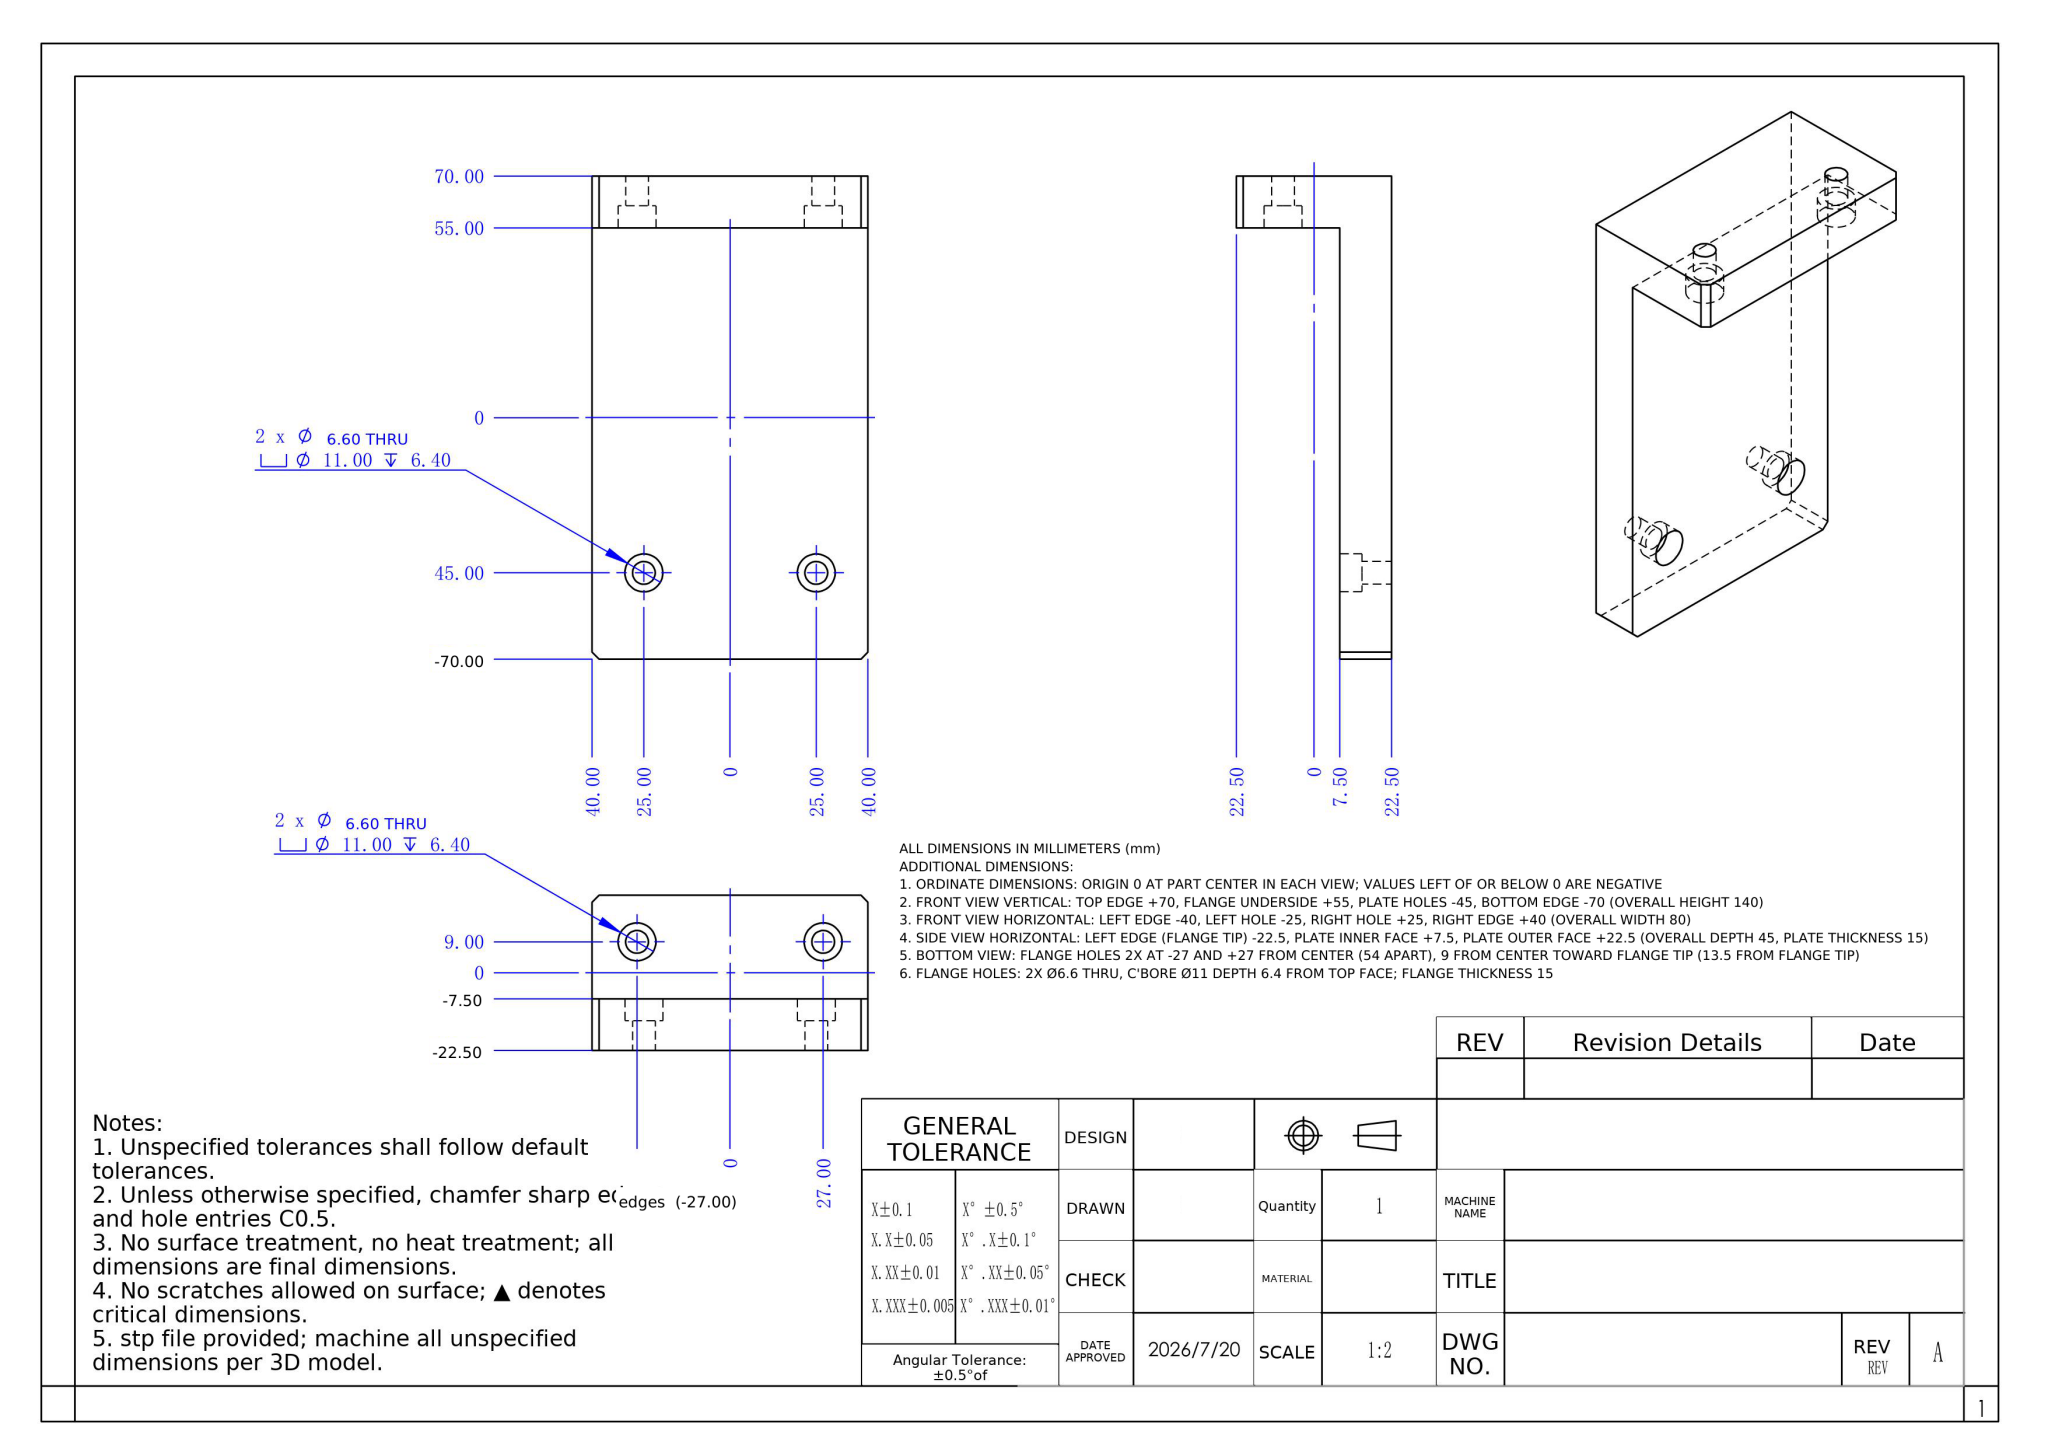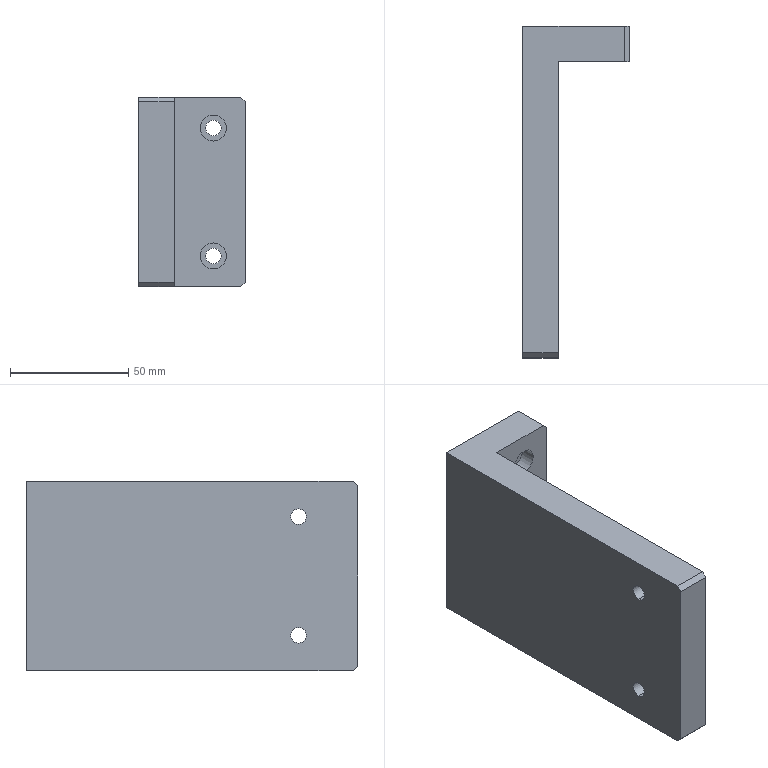Part | NX | mm | 1 solid | 32 faces | box 45 x 140 x 80 mm | volume 200270 mm3 | cylinder 16 | plane 16 | commonest cylinder face diameters 11 x8 6.6 x8
STEP:
#1=CARTESIAN_POINT('',(8.6,25.,20.5));
#2=VERTEX_POINT('',#1);
#3=CARTESIAN_POINT('',(8.6,25.,9.5));
#4=VERTEX_POINT('',#3);
#5=CARTESIAN_POINT('',(8.6,25.,15.));
#6=DIRECTION('',(1.,0.,0.));
#7=DIRECTION('',(0.,0.,-1.));
#8=AXIS2_PLACEMENT_3D('',#5,#6,#7);
#9=CIRCLE('',#8,5.5);
#10=EDGE_CURVE('',#2,#4,#9,.T.);
#11=ORIENTED_EDGE('',*,*,#10,.F.);
#12=CARTESIAN_POINT('',(15.,25.,20.5));
#13=VERTEX_POINT('',#12);
#14=CARTESIAN_POINT('',(15.,25.,20.5));
#15=DIRECTION('',(1.,0.,0.));
#16=VECTOR('',#15,1000.);
#17=LINE('',#14,#16);
#18=EDGE_CURVE('',#2,#13,#17,.T.);
#19=ORIENTED_EDGE('',*,*,#18,.T.);
#20=CARTESIAN_POINT('',(15.,25.,9.5));
#21=VERTEX_POINT('',#20);
#22=CARTESIAN_POINT('',(15.,25.,15.));
#23=DIRECTION('',(1.,0.,0.));
#24=DIRECTION('',(0.,0.,-1.));
#25=AXIS2_PLACEMENT_3D('',#22,#23,#24);
#26=CIRCLE('',#25,5.5);
#27=EDGE_CURVE('',#13,#21,#26,.T.);
#28=ORIENTED_EDGE('',*,*,#27,.T.);
#29=CARTESIAN_POINT('',(15.,25.,9.5));
#30=DIRECTION('',(1.,0.,0.));
#31=VECTOR('',#30,1000.);
#32=LINE('',#29,#31);
#33=EDGE_CURVE('',#4,#21,#32,.T.);
#34=ORIENTED_EDGE('',*,*,#33,.F.);
#35=EDGE_LOOP('',(#11,#19,#28,#34));
#36=FACE_OUTER_BOUND('',#35,.T.);
#37=CARTESIAN_POINT('',(15.,25.,15.));
#38=DIRECTION('',(1.,0.,0.));
#39=DIRECTION('',(0.,0.,-1.));
#40=AXIS2_PLACEMENT_3D('',#37,#38,#39);
#41=CYLINDRICAL_SURFACE('',#40,5.5);
#42=ADVANCED_FACE('',(#36),#41,.F.);
#43=CARTESIAN_POINT('',(0.,25.,18.3));
#44=VERTEX_POINT('',#43);
#45=CARTESIAN_POINT('',(0.,25.,11.7));
#46=VERTEX_POINT('',#45);
#47=CARTESIAN_POINT('',(0.,25.,15.));
#48=DIRECTION('',(1.,0.,0.));
#49=DIRECTION('',(0.,0.,-1.));
#50=AXIS2_PLACEMENT_3D('',#47,#48,#49);
#51=CIRCLE('',#50,3.3);
#52=EDGE_CURVE('',#44,#46,#51,.T.);
#53=ORIENTED_EDGE('',*,*,#52,.F.);
#54=CARTESIAN_POINT('',(8.6,25.,18.3));
#55=VERTEX_POINT('',#54);
#56=CARTESIAN_POINT('',(15.,25.,18.3));
#57=DIRECTION('',(1.,0.,0.));
#58=VECTOR('',#57,1000.);
#59=LINE('',#56,#58);
#60=EDGE_CURVE('',#44,#55,#59,.T.);
#61=ORIENTED_EDGE('',*,*,#60,.T.);
#62=CARTESIAN_POINT('',(8.6,25.,11.7));
#63=VERTEX_POINT('',#62);
#64=CARTESIAN_POINT('',(8.6,25.,15.));
#65=DIRECTION('',(1.,0.,0.));
#66=DIRECTION('',(0.,0.,-1.));
#67=AXIS2_PLACEMENT_3D('',#64,#65,#66);
#68=CIRCLE('',#67,3.3);
#69=EDGE_CURVE('',#55,#63,#68,.T.);
#70=ORIENTED_EDGE('',*,*,#69,.T.);
#71=CARTESIAN_POINT('',(15.,25.,11.7));
#72=DIRECTION('',(1.,0.,0.));
#73=VECTOR('',#72,1000.);
#74=LINE('',#71,#73);
#75=EDGE_CURVE('',#46,#63,#74,.T.);
#76=ORIENTED_EDGE('',*,*,#75,.F.);
#77=EDGE_LOOP('',(#53,#61,#70,#76));
#78=FACE_OUTER_BOUND('',#77,.T.);
#79=CARTESIAN_POINT('',(15.,25.,15.));
#80=DIRECTION('',(1.,0.,0.));
#81=DIRECTION('',(0.,0.,-1.));
#82=AXIS2_PLACEMENT_3D('',#79,#80,#81);
#83=CYLINDRICAL_SURFACE('',#82,3.3);
#84=ADVANCED_FACE('',(#78),#83,.F.);
#85=CARTESIAN_POINT('',(8.6,25.,70.5));
#86=VERTEX_POINT('',#85);
#87=CARTESIAN_POINT('',(8.6,25.,59.5));
#88=VERTEX_POINT('',#87);
#89=CARTESIAN_POINT('',(8.6,25.,65.));
#90=DIRECTION('',(1.,0.,0.));
#91=DIRECTION('',(0.,0.,-1.));
#92=AXIS2_PLACEMENT_3D('',#89,#90,#91);
#93=CIRCLE('',#92,5.5);
#94=EDGE_CURVE('',#86,#88,#93,.T.);
#95=ORIENTED_EDGE('',*,*,#94,.F.);
#96=CARTESIAN_POINT('',(15.,25.,70.5));
#97=VERTEX_POINT('',#96);
#98=CARTESIAN_POINT('',(15.,25.,70.5));
#99=DIRECTION('',(1.,0.,0.));
#100=VECTOR('',#99,1000.);
#101=LINE('',#98,#100);
#102=EDGE_CURVE('',#86,#97,#101,.T.);
#103=ORIENTED_EDGE('',*,*,#102,.T.);
#104=CARTESIAN_POINT('',(15.,25.,59.5));
#105=VERTEX_POINT('',#104);
#106=CARTESIAN_POINT('',(15.,25.,65.));
#107=DIRECTION('',(1.,0.,0.));
#108=DIRECTION('',(0.,0.,-1.));
#109=AXIS2_PLACEMENT_3D('',#106,#107,#108);
#110=CIRCLE('',#109,5.5);
#111=EDGE_CURVE('',#97,#105,#110,.T.);
#112=ORIENTED_EDGE('',*,*,#111,.T.);
#113=CARTESIAN_POINT('',(15.,25.,59.5));
#114=DIRECTION('',(1.,0.,0.));
#115=VECTOR('',#114,1000.);
#116=LINE('',#113,#115);
#117=EDGE_CURVE('',#88,#105,#116,.T.);
#118=ORIENTED_EDGE('',*,*,#117,.F.);
#119=EDGE_LOOP('',(#95,#103,#112,#118));
#120=FACE_OUTER_BOUND('',#119,.T.);
#121=CARTESIAN_POINT('',(15.,25.,65.));
#122=DIRECTION('',(1.,0.,0.));
#123=DIRECTION('',(0.,0.,-1.));
#124=AXIS2_PLACEMENT_3D('',#121,#122,#123);
#125=CYLINDRICAL_SURFACE('',#124,5.5);
#126=ADVANCED_FACE('',(#120),#125,.F.);
#127=CARTESIAN_POINT('',(0.,25.,68.3));
#128=VERTEX_POINT('',#127);
#129=CARTESIAN_POINT('',(0.,25.,61.7));
#130=VERTEX_POINT('',#129);
#131=CARTESIAN_POINT('',(0.,25.,65.));
#132=DIRECTION('',(1.,0.,0.));
#133=DIRECTION('',(0.,0.,-1.));
#134=AXIS2_PLACEMENT_3D('',#131,#132,#133);
#135=CIRCLE('',#134,3.3);
#136=EDGE_CURVE('',#128,#130,#135,.T.);
#137=ORIENTED_EDGE('',*,*,#136,.F.);
#138=CARTESIAN_POINT('',(8.6,25.,68.3));
#139=VERTEX_POINT('',#138);
#140=CARTESIAN_POINT('',(15.,25.,68.3));
#141=DIRECTION('',(1.,0.,0.));
#142=VECTOR('',#141,1000.);
#143=LINE('',#140,#142);
#144=EDGE_CURVE('',#128,#139,#143,.T.);
#145=ORIENTED_EDGE('',*,*,#144,.T.);
#146=CARTESIAN_POINT('',(8.6,25.,61.7));
#147=VERTEX_POINT('',#146);
#148=CARTESIAN_POINT('',(8.6,25.,65.));
#149=DIRECTION('',(1.,0.,0.));
#150=DIRECTION('',(0.,0.,-1.));
#151=AXIS2_PLACEMENT_3D('',#148,#149,#150);
#152=CIRCLE('',#151,3.3);
#153=EDGE_CURVE('',#139,#147,#152,.T.);
#154=ORIENTED_EDGE('',*,*,#153,.T.);
#155=CARTESIAN_POINT('',(15.,25.,61.7));
#156=DIRECTION('',(1.,0.,0.));
#157=VECTOR('',#156,1000.);
#158=LINE('',#155,#157);
#159=EDGE_CURVE('',#130,#147,#158,.T.);
#160=ORIENTED_EDGE('',*,*,#159,.F.);
#161=EDGE_LOOP('',(#137,#145,#154,#160));
#162=FACE_OUTER_BOUND('',#161,.T.);
#163=CARTESIAN_POINT('',(15.,25.,65.));
#164=DIRECTION('',(1.,0.,0.));
#165=DIRECTION('',(0.,0.,-1.));
#166=AXIS2_PLACEMENT_3D('',#163,#164,#165);
#167=CYLINDRICAL_SURFACE('',#166,3.3);
#168=ADVANCED_FACE('',(#162),#167,.F.);
#169=CARTESIAN_POINT('',(31.5,131.4,18.5));
#170=VERTEX_POINT('',#169);
#171=CARTESIAN_POINT('',(31.5,131.4,7.5));
#172=VERTEX_POINT('',#171);
#173=CARTESIAN_POINT('',(31.5,131.4,13.));
#174=DIRECTION('',(0.,-1.,0.));
#175=DIRECTION('',(0.,0.,-1.));
#176=AXIS2_PLACEMENT_3D('',#173,#174,#175);
#177=CIRCLE('',#176,5.5);
#178=EDGE_CURVE('',#170,#172,#177,.T.);
#179=ORIENTED_EDGE('',*,*,#178,.F.);
#180=CARTESIAN_POINT('',(31.5,125.,18.5));
#181=VERTEX_POINT('',#180);
#182=CARTESIAN_POINT('',(31.5,125.,18.5));
#183=DIRECTION('',(0.,-1.,0.));
#184=VECTOR('',#183,1000.);
#185=LINE('',#182,#184);
#186=EDGE_CURVE('',#170,#181,#185,.T.);
#187=ORIENTED_EDGE('',*,*,#186,.T.);
#188=CARTESIAN_POINT('',(31.5,125.,7.5));
#189=VERTEX_POINT('',#188);
#190=CARTESIAN_POINT('',(31.5,125.,13.));
#191=DIRECTION('',(0.,-1.,0.));
#192=DIRECTION('',(0.,0.,-1.));
#193=AXIS2_PLACEMENT_3D('',#190,#191,#192);
#194=CIRCLE('',#193,5.5);
#195=EDGE_CURVE('',#181,#189,#194,.T.);
#196=ORIENTED_EDGE('',*,*,#195,.T.);
#197=CARTESIAN_POINT('',(31.5,125.,7.5));
#198=DIRECTION('',(0.,-1.,0.));
#199=VECTOR('',#198,1000.);
#200=LINE('',#197,#199);
#201=EDGE_CURVE('',#172,#189,#200,.T.);
#202=ORIENTED_EDGE('',*,*,#201,.F.);
#203=EDGE_LOOP('',(#179,#187,#196,#202));
#204=FACE_OUTER_BOUND('',#203,.T.);
#205=CARTESIAN_POINT('',(31.5,125.,13.));
#206=DIRECTION('',(0.,-1.,0.));
#207=DIRECTION('',(0.,0.,-1.));
#208=AXIS2_PLACEMENT_3D('',#205,#206,#207);
#209=CYLINDRICAL_SURFACE('',#208,5.5);
#210=ADVANCED_FACE('',(#204),#209,.F.);
#211=CARTESIAN_POINT('',(31.5,140.,16.3));
#212=VERTEX_POINT('',#211);
#213=CARTESIAN_POINT('',(31.5,140.,9.7));
#214=VERTEX_POINT('',#213);
#215=CARTESIAN_POINT('',(31.5,140.,13.));
#216=DIRECTION('',(0.,-1.,0.));
#217=DIRECTION('',(0.,0.,-1.));
#218=AXIS2_PLACEMENT_3D('',#215,#216,#217);
#219=CIRCLE('',#218,3.3);
#220=EDGE_CURVE('',#212,#214,#219,.T.);
#221=ORIENTED_EDGE('',*,*,#220,.F.);
#222=CARTESIAN_POINT('',(31.5,131.4,16.3));
#223=VERTEX_POINT('',#222);
#224=CARTESIAN_POINT('',(31.5,125.,16.3));
#225=DIRECTION('',(0.,-1.,0.));
#226=VECTOR('',#225,1000.);
#227=LINE('',#224,#226);
#228=EDGE_CURVE('',#212,#223,#227,.T.);
#229=ORIENTED_EDGE('',*,*,#228,.T.);
#230=CARTESIAN_POINT('',(31.5,131.4,9.7));
#231=VERTEX_POINT('',#230);
#232=CARTESIAN_POINT('',(31.5,131.4,13.));
#233=DIRECTION('',(0.,-1.,0.));
#234=DIRECTION('',(0.,0.,-1.));
#235=AXIS2_PLACEMENT_3D('',#232,#233,#234);
#236=CIRCLE('',#235,3.3);
#237=EDGE_CURVE('',#223,#231,#236,.T.);
#238=ORIENTED_EDGE('',*,*,#237,.T.);
#239=CARTESIAN_POINT('',(31.5,125.,9.7));
#240=DIRECTION('',(0.,-1.,0.));
#241=VECTOR('',#240,1000.);
#242=LINE('',#239,#241);
#243=EDGE_CURVE('',#214,#231,#242,.T.);
#244=ORIENTED_EDGE('',*,*,#243,.F.);
#245=EDGE_LOOP('',(#221,#229,#238,#244));
#246=FACE_OUTER_BOUND('',#245,.T.);
#247=CARTESIAN_POINT('',(31.5,125.,13.));
#248=DIRECTION('',(0.,-1.,0.));
#249=DIRECTION('',(0.,0.,-1.));
#250=AXIS2_PLACEMENT_3D('',#247,#248,#249);
#251=CYLINDRICAL_SURFACE('',#250,3.3);
#252=ADVANCED_FACE('',(#246),#251,.F.);
#253=CARTESIAN_POINT('',(31.5,131.4,72.5));
#254=VERTEX_POINT('',#253);
#255=CARTESIAN_POINT('',(31.5,131.4,61.5));
#256=VERTEX_POINT('',#255);
#257=CARTESIAN_POINT('',(31.5,131.4,67.));
#258=DIRECTION('',(0.,-1.,0.));
#259=DIRECTION('',(0.,0.,-1.));
#260=AXIS2_PLACEMENT_3D('',#257,#258,#259);
#261=CIRCLE('',#260,5.5);
#262=EDGE_CURVE('',#254,#256,#261,.T.);
#263=ORIENTED_EDGE('',*,*,#262,.F.);
#264=CARTESIAN_POINT('',(31.5,125.,72.5));
#265=VERTEX_POINT('',#264);
#266=CARTESIAN_POINT('',(31.5,125.,72.5));
#267=DIRECTION('',(0.,-1.,0.));
#268=VECTOR('',#267,1000.);
#269=LINE('',#266,#268);
#270=EDGE_CURVE('',#254,#265,#269,.T.);
#271=ORIENTED_EDGE('',*,*,#270,.T.);
#272=CARTESIAN_POINT('',(31.5,125.,61.5));
#273=VERTEX_POINT('',#272);
#274=CARTESIAN_POINT('',(31.5,125.,67.));
#275=DIRECTION('',(0.,-1.,0.));
#276=DIRECTION('',(0.,0.,-1.));
#277=AXIS2_PLACEMENT_3D('',#274,#275,#276);
#278=CIRCLE('',#277,5.5);
#279=EDGE_CURVE('',#265,#273,#278,.T.);
#280=ORIENTED_EDGE('',*,*,#279,.T.);
#281=CARTESIAN_POINT('',(31.5,125.,61.5));
#282=DIRECTION('',(0.,-1.,0.));
#283=VECTOR('',#282,1000.);
#284=LINE('',#281,#283);
#285=EDGE_CURVE('',#256,#273,#284,.T.);
#286=ORIENTED_EDGE('',*,*,#285,.F.);
#287=EDGE_LOOP('',(#263,#271,#280,#286));
#288=FACE_OUTER_BOUND('',#287,.T.);
#289=CARTESIAN_POINT('',(31.5,125.,67.));
#290=DIRECTION('',(0.,-1.,0.));
#291=DIRECTION('',(0.,0.,-1.));
#292=AXIS2_PLACEMENT_3D('',#289,#290,#291);
#293=CYLINDRICAL_SURFACE('',#292,5.5);
#294=ADVANCED_FACE('',(#288),#293,.F.);
#295=CARTESIAN_POINT('',(31.5,140.,70.3));
#296=VERTEX_POINT('',#295);
#297=CARTESIAN_POINT('',(31.5,140.,63.7));
#298=VERTEX_POINT('',#297);
#299=CARTESIAN_POINT('',(31.5,140.,67.));
#300=DIRECTION('',(0.,-1.,0.));
#301=DIRECTION('',(0.,0.,-1.));
#302=AXIS2_PLACEMENT_3D('',#299,#300,#301);
#303=CIRCLE('',#302,3.3);
#304=EDGE_CURVE('',#296,#298,#303,.T.);
#305=ORIENTED_EDGE('',*,*,#304,.F.);
#306=CARTESIAN_POINT('',(31.5,131.4,70.3));
#307=VERTEX_POINT('',#306);
#308=CARTESIAN_POINT('',(31.5,125.,70.3));
#309=DIRECTION('',(0.,-1.,0.));
#310=VECTOR('',#309,1000.);
#311=LINE('',#308,#310);
#312=EDGE_CURVE('',#296,#307,#311,.T.);
#313=ORIENTED_EDGE('',*,*,#312,.T.);
#314=CARTESIAN_POINT('',(31.5,131.4,63.7));
#315=VERTEX_POINT('',#314);
#316=CARTESIAN_POINT('',(31.5,131.4,67.));
#317=DIRECTION('',(0.,-1.,0.));
#318=DIRECTION('',(0.,0.,-1.));
#319=AXIS2_PLACEMENT_3D('',#316,#317,#318);
#320=CIRCLE('',#319,3.3);
#321=EDGE_CURVE('',#307,#315,#320,.T.);
#322=ORIENTED_EDGE('',*,*,#321,.T.);
#323=CARTESIAN_POINT('',(31.5,125.,63.7));
#324=DIRECTION('',(0.,-1.,0.));
#325=VECTOR('',#324,1000.);
#326=LINE('',#323,#325);
#327=EDGE_CURVE('',#298,#315,#326,.T.);
#328=ORIENTED_EDGE('',*,*,#327,.F.);
#329=EDGE_LOOP('',(#305,#313,#322,#328));
#330=FACE_OUTER_BOUND('',#329,.T.);
#331=CARTESIAN_POINT('',(31.5,125.,67.));
#332=DIRECTION('',(0.,-1.,0.));
#333=DIRECTION('',(0.,0.,-1.));
#334=AXIS2_PLACEMENT_3D('',#331,#332,#333);
#335=CYLINDRICAL_SURFACE('',#334,3.3);
#336=ADVANCED_FACE('',(#330),#335,.F.);
#337=CARTESIAN_POINT('',(0.,2.,80.));
#338=VERTEX_POINT('',#337);
#339=CARTESIAN_POINT('',(0.,140.,80.));
#340=VERTEX_POINT('',#339);
#341=CARTESIAN_POINT('',(0.,0.,80.));
#342=DIRECTION('',(0.,1.,0.));
#343=VECTOR('',#342,1000.);
#344=LINE('',#341,#343);
#345=EDGE_CURVE('',#338,#340,#344,.T.);
#346=ORIENTED_EDGE('',*,*,#345,.F.);
#347=CARTESIAN_POINT('',(15.,2.,80.));
#348=VERTEX_POINT('',#347);
#349=CARTESIAN_POINT('',(0.,2.,80.));
#350=DIRECTION('',(1.,0.,0.));
#351=VECTOR('',#350,1000.);
#352=LINE('',#349,#351);
#353=EDGE_CURVE('',#338,#348,#352,.T.);
#354=ORIENTED_EDGE('',*,*,#353,.T.);
#355=CARTESIAN_POINT('',(15.,125.,80.));
#356=VERTEX_POINT('',#355);
#357=CARTESIAN_POINT('',(15.,0.,80.));
#358=DIRECTION('',(0.,1.,0.));
#359=VECTOR('',#358,1000.);
#360=LINE('',#357,#359);
#361=EDGE_CURVE('',#348,#356,#360,.T.);
#362=ORIENTED_EDGE('',*,*,#361,.T.);
#363=CARTESIAN_POINT('',(43.,125.,80.));
#364=VERTEX_POINT('',#363);
#365=CARTESIAN_POINT('',(15.,125.,80.));
#366=DIRECTION('',(1.,0.,0.));
#367=VECTOR('',#366,1000.);
#368=LINE('',#365,#367);
#369=EDGE_CURVE('',#356,#364,#368,.T.);
#370=ORIENTED_EDGE('',*,*,#369,.T.);
#371=CARTESIAN_POINT('',(43.,140.,80.));
#372=VERTEX_POINT('',#371);
#373=CARTESIAN_POINT('',(43.,140.,80.));
#374=DIRECTION('',(0.,1.,0.));
#375=VECTOR('',#374,1000.);
#376=LINE('',#373,#375);
#377=EDGE_CURVE('',#364,#372,#376,.T.);
#378=ORIENTED_EDGE('',*,*,#377,.T.);
#379=CARTESIAN_POINT('',(15.,140.,80.));
#380=DIRECTION('',(1.,0.,0.));
#381=VECTOR('',#380,1000.);
#382=LINE('',#379,#381);
#383=EDGE_CURVE('',#340,#372,#382,.T.);
#384=ORIENTED_EDGE('',*,*,#383,.F.);
#385=EDGE_LOOP('',(#346,#354,#362,#370,#378,#384));
#386=FACE_OUTER_BOUND('',#385,.T.);
#387=CARTESIAN_POINT('',(0.,0.,80.));
#388=DIRECTION('',(0.,0.,-1.));
#389=DIRECTION('',(-1.,0.,0.));
#390=AXIS2_PLACEMENT_3D('',#387,#388,#389);
#391=PLANE('',#390);
#392=ADVANCED_FACE('',(#386),#391,.F.);
#393=CARTESIAN_POINT('',(45.,140.,78.));
#394=VERTEX_POINT('',#393);
#395=CARTESIAN_POINT('',(45.,140.,2.));
#396=VERTEX_POINT('',#395);
#397=CARTESIAN_POINT('',(45.,140.,80.));
#398=DIRECTION('',(0.,0.,-1.));
#399=VECTOR('',#398,1000.);
#400=LINE('',#397,#399);
#401=EDGE_CURVE('',#394,#396,#400,.T.);
#402=ORIENTED_EDGE('',*,*,#401,.F.);
#403=CARTESIAN_POINT('',(45.,125.,78.));
#404=VERTEX_POINT('',#403);
#405=CARTESIAN_POINT('',(45.,125.,78.));
#406=DIRECTION('',(0.,-1.,0.));
#407=VECTOR('',#406,1000.);
#408=LINE('',#405,#407);
#409=EDGE_CURVE('',#394,#404,#408,.T.);
#410=ORIENTED_EDGE('',*,*,#409,.T.);
#411=CARTESIAN_POINT('',(45.,125.,2.));
#412=VERTEX_POINT('',#411);
#413=CARTESIAN_POINT('',(45.,125.,80.));
#414=DIRECTION('',(0.,0.,-1.));
#415=VECTOR('',#414,1000.);
#416=LINE('',#413,#415);
#417=EDGE_CURVE('',#404,#412,#416,.T.);
#418=ORIENTED_EDGE('',*,*,#417,.T.);
#419=CARTESIAN_POINT('',(45.,140.,2.));
#420=DIRECTION('',(0.,1.,0.));
#421=VECTOR('',#420,1000.);
#422=LINE('',#419,#421);
#423=EDGE_CURVE('',#412,#396,#422,.T.);
#424=ORIENTED_EDGE('',*,*,#423,.T.);
#425=EDGE_LOOP('',(#402,#410,#418,#424));
#426=FACE_OUTER_BOUND('',#425,.T.);
#427=CARTESIAN_POINT('',(45.,140.,80.));
#428=DIRECTION('',(1.,0.,0.));
#429=DIRECTION('',(0.,0.,-1.));
#430=AXIS2_PLACEMENT_3D('',#427,#428,#429);
#431=PLANE('',#430);
#432=ADVANCED_FACE('',(#426),#431,.T.);
#433=CARTESIAN_POINT('',(15.,2.,0.));
#434=VERTEX_POINT('',#433);
#435=CARTESIAN_POINT('',(15.,125.,0.));
#436=VERTEX_POINT('',#435);
#437=CARTESIAN_POINT('',(15.,0.,0.));
#438=DIRECTION('',(0.,1.,0.));
#439=VECTOR('',#438,1000.);
#440=LINE('',#437,#439);
#441=EDGE_CURVE('',#434,#436,#440,.T.);
#442=ORIENTED_EDGE('',*,*,#441,.F.);
#443=CARTESIAN_POINT('',(0.,2.,0.));
#444=VERTEX_POINT('',#443);
#445=CARTESIAN_POINT('',(0.,2.,0.));
#446=DIRECTION('',(-1.,0.,0.));
#447=VECTOR('',#446,1000.);
#448=LINE('',#445,#447);
#449=EDGE_CURVE('',#434,#444,#448,.T.);
#450=ORIENTED_EDGE('',*,*,#449,.T.);
#451=CARTESIAN_POINT('',(0.,140.,0.));
#452=VERTEX_POINT('',#451);
#453=CARTESIAN_POINT('',(0.,0.,0.));
#454=DIRECTION('',(0.,1.,0.));
#455=VECTOR('',#454,1000.);
#456=LINE('',#453,#455);
#457=EDGE_CURVE('',#444,#452,#456,.T.);
#458=ORIENTED_EDGE('',*,*,#457,.T.);
#459=CARTESIAN_POINT('',(43.,140.,0.));
#460=VERTEX_POINT('',#459);
#461=CARTESIAN_POINT('',(15.,140.,0.));
#462=DIRECTION('',(1.,0.,0.));
#463=VECTOR('',#462,1000.);
#464=LINE('',#461,#463);
#465=EDGE_CURVE('',#452,#460,#464,.T.);
#466=ORIENTED_EDGE('',*,*,#465,.T.);
#467=CARTESIAN_POINT('',(43.,125.,0.));
#468=VERTEX_POINT('',#467);
#469=CARTESIAN_POINT('',(43.,0.,0.));
#470=DIRECTION('',(0.,-1.,0.));
#471=VECTOR('',#470,1000.);
#472=LINE('',#469,#471);
#473=EDGE_CURVE('',#460,#468,#472,.T.);
#474=ORIENTED_EDGE('',*,*,#473,.T.);
#475=CARTESIAN_POINT('',(15.,125.,0.));
#476=DIRECTION('',(1.,0.,0.));
#477=VECTOR('',#476,1000.);
#478=LINE('',#475,#477);
#479=EDGE_CURVE('',#436,#468,#478,.T.);
#480=ORIENTED_EDGE('',*,*,#479,.F.);
#481=EDGE_LOOP('',(#442,#450,#458,#466,#474,#480));
#482=FACE_OUTER_BOUND('',#481,.T.);
#483=CARTESIAN_POINT('',(0.,0.,0.));
#484=DIRECTION('',(0.,0.,-1.));
#485=DIRECTION('',(-1.,0.,0.));
#486=AXIS2_PLACEMENT_3D('',#483,#484,#485);
#487=PLANE('',#486);
#488=ADVANCED_FACE('',(#482),#487,.T.);
#489=CARTESIAN_POINT('',(31.5,125.,13.));
#490=DIRECTION('',(0.,-1.,0.));
#491=DIRECTION('',(0.,0.,-1.));
#492=AXIS2_PLACEMENT_3D('',#489,#490,#491);
#493=CIRCLE('',#492,5.5);
#494=EDGE_CURVE('',#189,#181,#493,.T.);
#495=ORIENTED_EDGE('',*,*,#494,.F.);
#496=ORIENTED_EDGE('',*,*,#195,.F.);
#497=EDGE_LOOP('',(#495,#496));
#498=FACE_BOUND('',#497,.T.);
#499=CARTESIAN_POINT('',(31.5,125.,67.));
#500=DIRECTION('',(0.,-1.,0.));
#501=DIRECTION('',(0.,0.,-1.));
#502=AXIS2_PLACEMENT_3D('',#499,#500,#501);
#503=CIRCLE('',#502,5.5);
#504=EDGE_CURVE('',#273,#265,#503,.T.);
#505=ORIENTED_EDGE('',*,*,#504,.F.);
#506=ORIENTED_EDGE('',*,*,#279,.F.);
#507=EDGE_LOOP('',(#505,#506));
#508=FACE_BOUND('',#507,.T.);
#509=ORIENTED_EDGE('',*,*,#417,.F.);
#510=CARTESIAN_POINT('',(45.,125.,78.));
#511=DIRECTION('',(-0.7071,0.,0.7071));
#512=VECTOR('',#511,1000.);
#513=LINE('',#510,#512);
#514=EDGE_CURVE('',#404,#364,#513,.T.);
#515=ORIENTED_EDGE('',*,*,#514,.T.);
#516=ORIENTED_EDGE('',*,*,#369,.F.);
#517=CARTESIAN_POINT('',(15.,125.,80.));
#518=DIRECTION('',(0.,0.,-1.));
#519=VECTOR('',#518,1000.);
#520=LINE('',#517,#519);
#521=EDGE_CURVE('',#356,#436,#520,.T.);
#522=ORIENTED_EDGE('',*,*,#521,.T.);
#523=ORIENTED_EDGE('',*,*,#479,.T.);
#524=CARTESIAN_POINT('',(43.,125.,0.));
#525=DIRECTION('',(0.7071,0.,0.7071));
#526=VECTOR('',#525,1000.);
#527=LINE('',#524,#526);
#528=EDGE_CURVE('',#468,#412,#527,.T.);
#529=ORIENTED_EDGE('',*,*,#528,.T.);
#530=EDGE_LOOP('',(#509,#515,#516,#522,#523,#529));
#531=FACE_OUTER_BOUND('',#530,.T.);
#532=CARTESIAN_POINT('',(15.,125.,80.));
#533=DIRECTION('',(0.,1.,0.));
#534=DIRECTION('',(0.,0.,1.));
#535=AXIS2_PLACEMENT_3D('',#532,#533,#534);
#536=PLANE('',#535);
#537=ADVANCED_FACE('',(#498,#508,#531),#536,.F.);
#538=CARTESIAN_POINT('',(31.5,140.,13.));
#539=DIRECTION('',(0.,-1.,0.));
#540=DIRECTION('',(0.,0.,-1.));
#541=AXIS2_PLACEMENT_3D('',#538,#539,#540);
#542=CIRCLE('',#541,3.3);
#543=EDGE_CURVE('',#214,#212,#542,.T.);
#544=ORIENTED_EDGE('',*,*,#543,.T.);
#545=ORIENTED_EDGE('',*,*,#220,.T.);
#546=EDGE_LOOP('',(#544,#545));
#547=FACE_BOUND('',#546,.T.);
#548=CARTESIAN_POINT('',(31.5,140.,67.));
#549=DIRECTION('',(0.,-1.,0.));
#550=DIRECTION('',(0.,0.,-1.));
#551=AXIS2_PLACEMENT_3D('',#548,#549,#550);
#552=CIRCLE('',#551,3.3);
#553=EDGE_CURVE('',#298,#296,#552,.T.);
#554=ORIENTED_EDGE('',*,*,#553,.T.);
#555=ORIENTED_EDGE('',*,*,#304,.T.);
#556=EDGE_LOOP('',(#554,#555));
#557=FACE_BOUND('',#556,.T.);
#558=ORIENTED_EDGE('',*,*,#383,.T.);
#559=CARTESIAN_POINT('',(29.,140.,94.));
#560=DIRECTION('',(0.7071,0.,-0.7071));
#561=VECTOR('',#560,1000.);
#562=LINE('',#559,#561);
#563=EDGE_CURVE('',#372,#394,#562,.T.);
#564=ORIENTED_EDGE('',*,*,#563,.T.);
#565=ORIENTED_EDGE('',*,*,#401,.T.);
#566=CARTESIAN_POINT('',(69.,140.,26.));
#567=DIRECTION('',(-0.7071,0.,-0.7071));
#568=VECTOR('',#567,1000.);
#569=LINE('',#566,#568);
#570=EDGE_CURVE('',#396,#460,#569,.T.);
#571=ORIENTED_EDGE('',*,*,#570,.T.);
#572=ORIENTED_EDGE('',*,*,#465,.F.);
#573=CARTESIAN_POINT('',(0.,140.,80.));
#574=DIRECTION('',(0.,0.,-1.));
#575=VECTOR('',#574,1000.);
#576=LINE('',#573,#575);
#577=EDGE_CURVE('',#340,#452,#576,.T.);
#578=ORIENTED_EDGE('',*,*,#577,.F.);
#579=EDGE_LOOP('',(#558,#564,#565,#571,#572,#578));
#580=FACE_OUTER_BOUND('',#579,.T.);
#581=CARTESIAN_POINT('',(15.,140.,80.));
#582=DIRECTION('',(0.,1.,0.));
#583=DIRECTION('',(0.,0.,1.));
#584=AXIS2_PLACEMENT_3D('',#581,#582,#583);
#585=PLANE('',#584);
#586=ADVANCED_FACE('',(#547,#557,#580),#585,.T.);
#587=CARTESIAN_POINT('',(0.,25.,15.));
#588=DIRECTION('',(1.,0.,0.));
#589=DIRECTION('',(0.,0.,-1.));
#590=AXIS2_PLACEMENT_3D('',#587,#588,#589);
#591=CIRCLE('',#590,3.3);
#592=EDGE_CURVE('',#46,#44,#591,.T.);
#593=ORIENTED_EDGE('',*,*,#592,.T.);
#594=ORIENTED_EDGE('',*,*,#52,.T.);
#595=EDGE_LOOP('',(#593,#594));
#596=FACE_BOUND('',#595,.T.);
#597=CARTESIAN_POINT('',(0.,25.,65.));
#598=DIRECTION('',(1.,0.,0.));
#599=DIRECTION('',(0.,0.,-1.));
#600=AXIS2_PLACEMENT_3D('',#597,#598,#599);
#601=CIRCLE('',#600,3.3);
#602=EDGE_CURVE('',#130,#128,#601,.T.);
#603=ORIENTED_EDGE('',*,*,#602,.T.);
#604=ORIENTED_EDGE('',*,*,#136,.T.);
#605=EDGE_LOOP('',(#603,#604));
#606=FACE_BOUND('',#605,.T.);
#607=ORIENTED_EDGE('',*,*,#457,.F.);
#608=CARTESIAN_POINT('',(0.,0.,2.));
#609=VERTEX_POINT('',#608);
#610=CARTESIAN_POINT('',(0.,-39.,41.));
#611=DIRECTION('',(0.,-0.7071,0.7071));
#612=VECTOR('',#611,1000.);
#613=LINE('',#610,#612);
#614=EDGE_CURVE('',#444,#609,#613,.T.);
#615=ORIENTED_EDGE('',*,*,#614,.T.);
#616=CARTESIAN_POINT('',(0.,0.,78.));
#617=VERTEX_POINT('',#616);
#618=CARTESIAN_POINT('',(0.,0.,80.));
#619=DIRECTION('',(0.,0.,-1.));
#620=VECTOR('',#619,1000.);
#621=LINE('',#618,#620);
#622=EDGE_CURVE('',#617,#609,#621,.T.);
#623=ORIENTED_EDGE('',*,*,#622,.F.);
#624=CARTESIAN_POINT('',(0.,1.,79.));
#625=DIRECTION('',(0.,0.7071,0.7071));
#626=VECTOR('',#625,1000.);
#627=LINE('',#624,#626);
#628=EDGE_CURVE('',#617,#338,#627,.T.);
#629=ORIENTED_EDGE('',*,*,#628,.T.);
#630=ORIENTED_EDGE('',*,*,#345,.T.);
#631=ORIENTED_EDGE('',*,*,#577,.T.);
#632=EDGE_LOOP('',(#607,#615,#623,#629,#630,#631));
#633=FACE_OUTER_BOUND('',#632,.T.);
#634=CARTESIAN_POINT('',(0.,0.,80.));
#635=DIRECTION('',(-1.,0.,0.));
#636=DIRECTION('',(0.,0.,1.));
#637=AXIS2_PLACEMENT_3D('',#634,#635,#636);
#638=PLANE('',#637);
#639=ADVANCED_FACE('',(#596,#606,#633),#638,.T.);
#640=ORIENTED_EDGE('',*,*,#622,.T.);
#641=CARTESIAN_POINT('',(15.,0.,2.));
#642=VERTEX_POINT('',#641);
#643=CARTESIAN_POINT('',(15.,0.,2.));
#644=DIRECTION('',(1.,0.,0.));
#645=VECTOR('',#644,1000.);
#646=LINE('',#643,#645);
#647=EDGE_CURVE('',#609,#642,#646,.T.);
#648=ORIENTED_EDGE('',*,*,#647,.T.);
#649=CARTESIAN_POINT('',(15.,0.,78.));
#650=VERTEX_POINT('',#649);
#651=CARTESIAN_POINT('',(15.,0.,80.));
#652=DIRECTION('',(0.,0.,-1.));
#653=VECTOR('',#652,1000.);
#654=LINE('',#651,#653);
#655=EDGE_CURVE('',#650,#642,#654,.T.);
#656=ORIENTED_EDGE('',*,*,#655,.F.);
#657=CARTESIAN_POINT('',(0.,0.,78.));
#658=DIRECTION('',(-1.,0.,0.));
#659=VECTOR('',#658,1000.);
#660=LINE('',#657,#659);
#661=EDGE_CURVE('',#650,#617,#660,.T.);
#662=ORIENTED_EDGE('',*,*,#661,.T.);
#663=EDGE_LOOP('',(#640,#648,#656,#662));
#664=FACE_OUTER_BOUND('',#663,.T.);
#665=CARTESIAN_POINT('',(0.,0.,80.));
#666=DIRECTION('',(0.,1.,0.));
#667=DIRECTION('',(0.,0.,1.));
#668=AXIS2_PLACEMENT_3D('',#665,#666,#667);
#669=PLANE('',#668);
#670=ADVANCED_FACE('',(#664),#669,.F.);
#671=CARTESIAN_POINT('',(15.,25.,15.));
#672=DIRECTION('',(1.,0.,0.));
#673=DIRECTION('',(0.,0.,-1.));
#674=AXIS2_PLACEMENT_3D('',#671,#672,#673);
#675=CIRCLE('',#674,5.5);
#676=EDGE_CURVE('',#21,#13,#675,.T.);
#677=ORIENTED_EDGE('',*,*,#676,.F.);
#678=ORIENTED_EDGE('',*,*,#27,.F.);
#679=EDGE_LOOP('',(#677,#678));
#680=FACE_BOUND('',#679,.T.);
#681=CARTESIAN_POINT('',(15.,25.,65.));
#682=DIRECTION('',(1.,0.,0.));
#683=DIRECTION('',(0.,0.,-1.));
#684=AXIS2_PLACEMENT_3D('',#681,#682,#683);
#685=CIRCLE('',#684,5.5);
#686=EDGE_CURVE('',#105,#97,#685,.T.);
#687=ORIENTED_EDGE('',*,*,#686,.F.);
#688=ORIENTED_EDGE('',*,*,#111,.F.);
#689=EDGE_LOOP('',(#687,#688));
#690=FACE_BOUND('',#689,.T.);
#691=ORIENTED_EDGE('',*,*,#655,.T.);
#692=CARTESIAN_POINT('',(15.,-0.,2.));
#693=DIRECTION('',(0.,0.7071,-0.7071));
#694=VECTOR('',#693,1000.);
#695=LINE('',#692,#694);
#696=EDGE_CURVE('',#642,#434,#695,.T.);
#697=ORIENTED_EDGE('',*,*,#696,.T.);
#698=ORIENTED_EDGE('',*,*,#441,.T.);
#699=ORIENTED_EDGE('',*,*,#521,.F.);
#700=ORIENTED_EDGE('',*,*,#361,.F.);
#701=CARTESIAN_POINT('',(15.,2.,80.));
#702=DIRECTION('',(-0.,-0.7071,-0.7071));
#703=VECTOR('',#702,1000.);
#704=LINE('',#701,#703);
#705=EDGE_CURVE('',#348,#650,#704,.T.);
#706=ORIENTED_EDGE('',*,*,#705,.T.);
#707=EDGE_LOOP('',(#691,#697,#698,#699,#700,#706));
#708=FACE_OUTER_BOUND('',#707,.T.);
#709=CARTESIAN_POINT('',(15.,0.,80.));
#710=DIRECTION('',(-1.,0.,0.));
#711=DIRECTION('',(-0.,-1.,0.));
#712=AXIS2_PLACEMENT_3D('',#709,#710,#711);
#713=PLANE('',#712);
#714=ADVANCED_FACE('',(#680,#690,#708),#713,.F.);
#715=ORIENTED_EDGE('',*,*,#563,.F.);
#716=ORIENTED_EDGE('',*,*,#377,.F.);
#717=ORIENTED_EDGE('',*,*,#514,.F.);
#718=ORIENTED_EDGE('',*,*,#409,.F.);
#719=EDGE_LOOP('',(#715,#716,#717,#718));
#720=FACE_OUTER_BOUND('',#719,.T.);
#721=CARTESIAN_POINT('',(45.,140.,78.));
#722=DIRECTION('',(0.7071,0.,0.7071));
#723=DIRECTION('',(0.,1.,0.));
#724=AXIS2_PLACEMENT_3D('',#721,#722,#723);
#725=PLANE('',#724);
#726=ADVANCED_FACE('',(#720),#725,.T.);
#727=ORIENTED_EDGE('',*,*,#570,.F.);
#728=ORIENTED_EDGE('',*,*,#423,.F.);
#729=ORIENTED_EDGE('',*,*,#528,.F.);
#730=ORIENTED_EDGE('',*,*,#473,.F.);
#731=EDGE_LOOP('',(#727,#728,#729,#730));
#732=FACE_OUTER_BOUND('',#731,.T.);
#733=CARTESIAN_POINT('',(43.,0.,0.));
#734=DIRECTION('',(-0.7071,0.,0.7071));
#735=DIRECTION('',(0.,-1.,0.));
#736=AXIS2_PLACEMENT_3D('',#733,#734,#735);
#737=PLANE('',#736);
#738=ADVANCED_FACE('',(#732),#737,.F.);
#739=ORIENTED_EDGE('',*,*,#614,.F.);
#740=ORIENTED_EDGE('',*,*,#449,.F.);
#741=ORIENTED_EDGE('',*,*,#696,.F.);
#742=ORIENTED_EDGE('',*,*,#647,.F.);
#743=EDGE_LOOP('',(#739,#740,#741,#742));
#744=FACE_OUTER_BOUND('',#743,.T.);
#745=CARTESIAN_POINT('',(0.,0.,2.));
#746=DIRECTION('',(0.,-0.7071,-0.7071));
#747=DIRECTION('',(-1.,0.,0.));
#748=AXIS2_PLACEMENT_3D('',#745,#746,#747);
#749=PLANE('',#748);
#750=ADVANCED_FACE('',(#744),#749,.T.);
#751=ORIENTED_EDGE('',*,*,#628,.F.);
#752=ORIENTED_EDGE('',*,*,#661,.F.);
#753=ORIENTED_EDGE('',*,*,#705,.F.);
#754=ORIENTED_EDGE('',*,*,#353,.F.);
#755=EDGE_LOOP('',(#751,#752,#753,#754));
#756=FACE_OUTER_BOUND('',#755,.T.);
#757=CARTESIAN_POINT('',(0.,2.,80.));
#758=DIRECTION('',(0.,0.7071,-0.7071));
#759=DIRECTION('',(1.,0.,0.));
#760=AXIS2_PLACEMENT_3D('',#757,#758,#759);
#761=PLANE('',#760);
#762=ADVANCED_FACE('',(#756),#761,.F.);
#763=ORIENTED_EDGE('',*,*,#312,.F.);
#764=ORIENTED_EDGE('',*,*,#553,.F.);
#765=ORIENTED_EDGE('',*,*,#327,.T.);
#766=CARTESIAN_POINT('',(31.5,131.4,67.));
#767=DIRECTION('',(0.,-1.,0.));
#768=DIRECTION('',(0.,0.,-1.));
#769=AXIS2_PLACEMENT_3D('',#766,#767,#768);
#770=CIRCLE('',#769,3.3);
#771=EDGE_CURVE('',#315,#307,#770,.T.);
#772=ORIENTED_EDGE('',*,*,#771,.T.);
#773=EDGE_LOOP('',(#763,#764,#765,#772));
#774=FACE_OUTER_BOUND('',#773,.T.);
#775=CARTESIAN_POINT('',(31.5,125.,67.));
#776=DIRECTION('',(0.,-1.,0.));
#777=DIRECTION('',(0.,0.,-1.));
#778=AXIS2_PLACEMENT_3D('',#775,#776,#777);
#779=CYLINDRICAL_SURFACE('',#778,3.3);
#780=ADVANCED_FACE('',(#774),#779,.F.);
#781=ORIENTED_EDGE('',*,*,#771,.F.);
#782=ORIENTED_EDGE('',*,*,#321,.F.);
#783=EDGE_LOOP('',(#781,#782));
#784=FACE_BOUND('',#783,.T.);
#785=CARTESIAN_POINT('',(31.5,131.4,67.));
#786=DIRECTION('',(0.,-1.,0.));
#787=DIRECTION('',(0.,0.,-1.));
#788=AXIS2_PLACEMENT_3D('',#785,#786,#787);
#789=CIRCLE('',#788,5.5);
#790=EDGE_CURVE('',#256,#254,#789,.T.);
#791=ORIENTED_EDGE('',*,*,#790,.T.);
#792=ORIENTED_EDGE('',*,*,#262,.T.);
#793=EDGE_LOOP('',(#791,#792));
#794=FACE_OUTER_BOUND('',#793,.T.);
#795=CARTESIAN_POINT('',(34.8,131.4,67.));
#796=DIRECTION('',(0.,1.,0.));
#797=DIRECTION('',(0.,0.,1.));
#798=AXIS2_PLACEMENT_3D('',#795,#796,#797);
#799=PLANE('',#798);
#800=ADVANCED_FACE('',(#784,#794),#799,.F.);
#801=ORIENTED_EDGE('',*,*,#270,.F.);
#802=ORIENTED_EDGE('',*,*,#790,.F.);
#803=ORIENTED_EDGE('',*,*,#285,.T.);
#804=ORIENTED_EDGE('',*,*,#504,.T.);
#805=EDGE_LOOP('',(#801,#802,#803,#804));
#806=FACE_OUTER_BOUND('',#805,.T.);
#807=CARTESIAN_POINT('',(31.5,125.,67.));
#808=DIRECTION('',(0.,-1.,0.));
#809=DIRECTION('',(0.,0.,-1.));
#810=AXIS2_PLACEMENT_3D('',#807,#808,#809);
#811=CYLINDRICAL_SURFACE('',#810,5.5);
#812=ADVANCED_FACE('',(#806),#811,.F.);
#813=ORIENTED_EDGE('',*,*,#228,.F.);
#814=ORIENTED_EDGE('',*,*,#543,.F.);
#815=ORIENTED_EDGE('',*,*,#243,.T.);
#816=CARTESIAN_POINT('',(31.5,131.4,13.));
#817=DIRECTION('',(0.,-1.,0.));
#818=DIRECTION('',(0.,0.,-1.));
#819=AXIS2_PLACEMENT_3D('',#816,#817,#818);
#820=CIRCLE('',#819,3.3);
#821=EDGE_CURVE('',#231,#223,#820,.T.);
#822=ORIENTED_EDGE('',*,*,#821,.T.);
#823=EDGE_LOOP('',(#813,#814,#815,#822));
#824=FACE_OUTER_BOUND('',#823,.T.);
#825=CARTESIAN_POINT('',(31.5,125.,13.));
#826=DIRECTION('',(0.,-1.,0.));
#827=DIRECTION('',(0.,0.,-1.));
#828=AXIS2_PLACEMENT_3D('',#825,#826,#827);
#829=CYLINDRICAL_SURFACE('',#828,3.3);
#830=ADVANCED_FACE('',(#824),#829,.F.);
#831=ORIENTED_EDGE('',*,*,#821,.F.);
#832=ORIENTED_EDGE('',*,*,#237,.F.);
#833=EDGE_LOOP('',(#831,#832));
#834=FACE_BOUND('',#833,.T.);
#835=CARTESIAN_POINT('',(31.5,131.4,13.));
#836=DIRECTION('',(0.,-1.,0.));
#837=DIRECTION('',(0.,0.,-1.));
#838=AXIS2_PLACEMENT_3D('',#835,#836,#837);
#839=CIRCLE('',#838,5.5);
#840=EDGE_CURVE('',#172,#170,#839,.T.);
#841=ORIENTED_EDGE('',*,*,#840,.T.);
#842=ORIENTED_EDGE('',*,*,#178,.T.);
#843=EDGE_LOOP('',(#841,#842));
#844=FACE_OUTER_BOUND('',#843,.T.);
#845=CARTESIAN_POINT('',(34.8,131.4,13.));
#846=DIRECTION('',(0.,1.,0.));
#847=DIRECTION('',(0.,0.,1.));
#848=AXIS2_PLACEMENT_3D('',#845,#846,#847);
#849=PLANE('',#848);
#850=ADVANCED_FACE('',(#834,#844),#849,.F.);
#851=ORIENTED_EDGE('',*,*,#186,.F.);
#852=ORIENTED_EDGE('',*,*,#840,.F.);
#853=ORIENTED_EDGE('',*,*,#201,.T.);
#854=ORIENTED_EDGE('',*,*,#494,.T.);
#855=EDGE_LOOP('',(#851,#852,#853,#854));
#856=FACE_OUTER_BOUND('',#855,.T.);
#857=CARTESIAN_POINT('',(31.5,125.,13.));
#858=DIRECTION('',(0.,-1.,0.));
#859=DIRECTION('',(0.,0.,-1.));
#860=AXIS2_PLACEMENT_3D('',#857,#858,#859);
#861=CYLINDRICAL_SURFACE('',#860,5.5);
#862=ADVANCED_FACE('',(#856),#861,.F.);
#863=ORIENTED_EDGE('',*,*,#144,.F.);
#864=ORIENTED_EDGE('',*,*,#602,.F.);
#865=ORIENTED_EDGE('',*,*,#159,.T.);
#866=CARTESIAN_POINT('',(8.6,25.,65.));
#867=DIRECTION('',(1.,0.,0.));
#868=DIRECTION('',(0.,0.,-1.));
#869=AXIS2_PLACEMENT_3D('',#866,#867,#868);
#870=CIRCLE('',#869,3.3);
#871=EDGE_CURVE('',#147,#139,#870,.T.);
#872=ORIENTED_EDGE('',*,*,#871,.T.);
#873=EDGE_LOOP('',(#863,#864,#865,#872));
#874=FACE_OUTER_BOUND('',#873,.T.);
#875=CARTESIAN_POINT('',(15.,25.,65.));
#876=DIRECTION('',(1.,0.,0.));
#877=DIRECTION('',(0.,0.,-1.));
#878=AXIS2_PLACEMENT_3D('',#875,#876,#877);
#879=CYLINDRICAL_SURFACE('',#878,3.3);
#880=ADVANCED_FACE('',(#874),#879,.F.);
#881=ORIENTED_EDGE('',*,*,#871,.F.);
#882=ORIENTED_EDGE('',*,*,#153,.F.);
#883=EDGE_LOOP('',(#881,#882));
#884=FACE_BOUND('',#883,.T.);
#885=CARTESIAN_POINT('',(8.6,25.,65.));
#886=DIRECTION('',(1.,0.,0.));
#887=DIRECTION('',(0.,0.,-1.));
#888=AXIS2_PLACEMENT_3D('',#885,#886,#887);
#889=CIRCLE('',#888,5.5);
#890=EDGE_CURVE('',#88,#86,#889,.T.);
#891=ORIENTED_EDGE('',*,*,#890,.T.);
#892=ORIENTED_EDGE('',*,*,#94,.T.);
#893=EDGE_LOOP('',(#891,#892));
#894=FACE_OUTER_BOUND('',#893,.T.);
#895=CARTESIAN_POINT('',(8.6,28.3,65.));
#896=DIRECTION('',(-1.,0.,0.));
#897=DIRECTION('',(0.,0.,1.));
#898=AXIS2_PLACEMENT_3D('',#895,#896,#897);
#899=PLANE('',#898);
#900=ADVANCED_FACE('',(#884,#894),#899,.F.);
#901=ORIENTED_EDGE('',*,*,#102,.F.);
#902=ORIENTED_EDGE('',*,*,#890,.F.);
#903=ORIENTED_EDGE('',*,*,#117,.T.);
#904=ORIENTED_EDGE('',*,*,#686,.T.);
#905=EDGE_LOOP('',(#901,#902,#903,#904));
#906=FACE_OUTER_BOUND('',#905,.T.);
#907=CARTESIAN_POINT('',(15.,25.,65.));
#908=DIRECTION('',(1.,0.,0.));
#909=DIRECTION('',(0.,0.,-1.));
#910=AXIS2_PLACEMENT_3D('',#907,#908,#909);
#911=CYLINDRICAL_SURFACE('',#910,5.5);
#912=ADVANCED_FACE('',(#906),#911,.F.);
#913=ORIENTED_EDGE('',*,*,#60,.F.);
#914=ORIENTED_EDGE('',*,*,#592,.F.);
#915=ORIENTED_EDGE('',*,*,#75,.T.);
#916=CARTESIAN_POINT('',(8.6,25.,15.));
#917=DIRECTION('',(1.,0.,0.));
#918=DIRECTION('',(0.,0.,-1.));
#919=AXIS2_PLACEMENT_3D('',#916,#917,#918);
#920=CIRCLE('',#919,3.3);
#921=EDGE_CURVE('',#63,#55,#920,.T.);
#922=ORIENTED_EDGE('',*,*,#921,.T.);
#923=EDGE_LOOP('',(#913,#914,#915,#922));
#924=FACE_OUTER_BOUND('',#923,.T.);
#925=CARTESIAN_POINT('',(15.,25.,15.));
#926=DIRECTION('',(1.,0.,0.));
#927=DIRECTION('',(0.,0.,-1.));
#928=AXIS2_PLACEMENT_3D('',#925,#926,#927);
#929=CYLINDRICAL_SURFACE('',#928,3.3);
#930=ADVANCED_FACE('',(#924),#929,.F.);
#931=ORIENTED_EDGE('',*,*,#921,.F.);
#932=ORIENTED_EDGE('',*,*,#69,.F.);
#933=EDGE_LOOP('',(#931,#932));
#934=FACE_BOUND('',#933,.T.);
#935=CARTESIAN_POINT('',(8.6,25.,15.));
#936=DIRECTION('',(1.,0.,0.));
#937=DIRECTION('',(0.,0.,-1.));
#938=AXIS2_PLACEMENT_3D('',#935,#936,#937);
#939=CIRCLE('',#938,5.5);
#940=EDGE_CURVE('',#4,#2,#939,.T.);
#941=ORIENTED_EDGE('',*,*,#940,.T.);
#942=ORIENTED_EDGE('',*,*,#10,.T.);
#943=EDGE_LOOP('',(#941,#942));
#944=FACE_OUTER_BOUND('',#943,.T.);
#945=CARTESIAN_POINT('',(8.6,28.3,15.));
#946=DIRECTION('',(-1.,0.,0.));
#947=DIRECTION('',(0.,0.,1.));
#948=AXIS2_PLACEMENT_3D('',#945,#946,#947);
#949=PLANE('',#948);
#950=ADVANCED_FACE('',(#934,#944),#949,.F.);
#951=ORIENTED_EDGE('',*,*,#18,.F.);
#952=ORIENTED_EDGE('',*,*,#940,.F.);
#953=ORIENTED_EDGE('',*,*,#33,.T.);
#954=ORIENTED_EDGE('',*,*,#676,.T.);
#955=EDGE_LOOP('',(#951,#952,#953,#954));
#956=FACE_OUTER_BOUND('',#955,.T.);
#957=CARTESIAN_POINT('',(15.,25.,15.));
#958=DIRECTION('',(1.,0.,0.));
#959=DIRECTION('',(0.,0.,-1.));
#960=AXIS2_PLACEMENT_3D('',#957,#958,#959);
#961=CYLINDRICAL_SURFACE('',#960,5.5);
#962=ADVANCED_FACE('',(#956),#961,.F.);
#963=CLOSED_SHELL('',(#42,#84,#126,#168,#210,#252,#294,#336,#392,#432,#488,#537,#586,#639,#670,#714,#726,#738,#750,#762,#780,#800,#812,#830,#850,#862,#880,#900,#912,#930,#950,#962));
#964=MANIFOLD_SOLID_BREP('',#963);
#965=CARTESIAN_POINT('',(0.,0.,0.));
#966=DIRECTION('',(0.,0.,1.));
#967=DIRECTION('',(1.,0.,0.));
#968=AXIS2_PLACEMENT_3D('',#965,#966,#967);
#969=(LENGTH_UNIT()NAMED_UNIT(*)SI_UNIT(.MILLI.,.METRE.));
#970=UNCERTAINTY_MEASURE_WITH_UNIT(LENGTH_MEASURE(0.00001),#969,'','');
#971=(NAMED_UNIT(*)PLANE_ANGLE_UNIT()SI_UNIT($,.RADIAN.));
#972=(NAMED_UNIT(*)SI_UNIT($,.STERADIAN.)SOLID_ANGLE_UNIT());
#973=(GEOMETRIC_REPRESENTATION_CONTEXT(3)GLOBAL_UNCERTAINTY_ASSIGNED_CONTEXT((#970))GLOBAL_UNIT_ASSIGNED_CONTEXT((#969,#971,#972))REPRESENTATION_CONTEXT('',''));
#974=ADVANCED_BREP_SHAPE_REPRESENTATION('',(#964,#968),#973);
#975=COLOUR_RGB('',0.7922,0.8196,0.9333);
#976=FILL_AREA_STYLE_COLOUR('',#975);
#977=FILL_AREA_STYLE('',(#976));
#978=SURFACE_STYLE_FILL_AREA(#977);
#979=SURFACE_SIDE_STYLE('',(#978));
#980=SURFACE_STYLE_USAGE(.BOTH.,#979);
#981=PRESENTATION_STYLE_ASSIGNMENT((#980));
#982=STYLED_ITEM('',(#981),#964);
#983=(LENGTH_UNIT()NAMED_UNIT(*)SI_UNIT(.MILLI.,.METRE.));
#984=UNCERTAINTY_MEASURE_WITH_UNIT(LENGTH_MEASURE(0.00001),#983,'','');
#985=(NAMED_UNIT(*)PLANE_ANGLE_UNIT()SI_UNIT($,.RADIAN.));
#986=(NAMED_UNIT(*)SI_UNIT($,.STERADIAN.)SOLID_ANGLE_UNIT());
#987=(GEOMETRIC_REPRESENTATION_CONTEXT(3)GLOBAL_UNCERTAINTY_ASSIGNED_CONTEXT((#984))GLOBAL_UNIT_ASSIGNED_CONTEXT((#983,#985,#986))REPRESENTATION_CONTEXT('',''));
#988=MECHANICAL_DESIGN_GEOMETRIC_PRESENTATION_REPRESENTATION('',(#982),#987);
#989=PRESENTATION_LAYER_ASSIGNMENT('','',(#982));